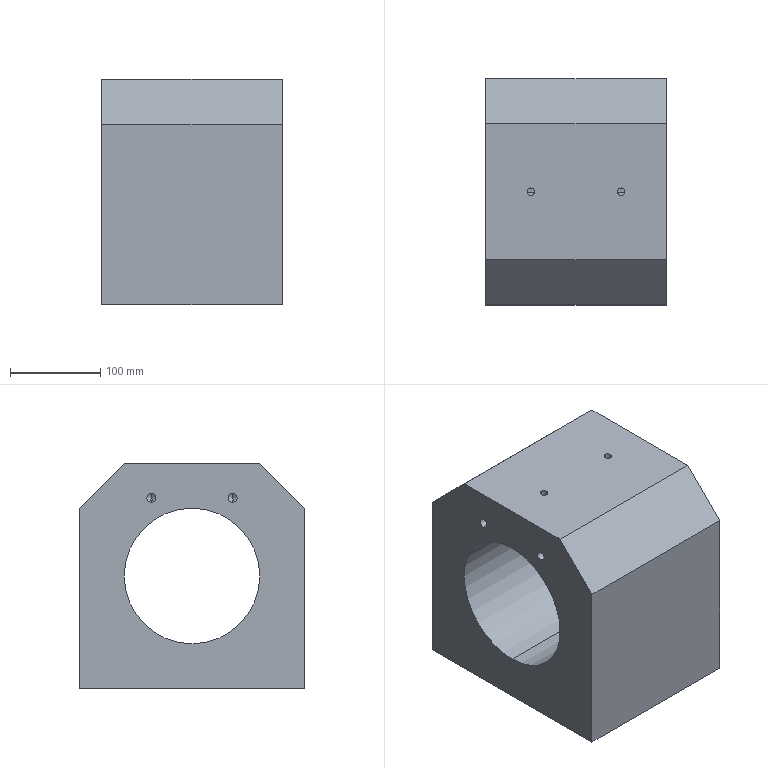Component | SolidWorks | BearingHousing-1_BearingHousing-1 | 1 solid | 30 faces | box 200 x 250 x 250 mm | volume 8448175 mm3 | cylinder 14 | cone 8 | plane 8 | commonest cylinder face diameters 10.2 x8 8.5 x4 150 x2 | material Plain Carbon Steel
STEP:
#1=COLOUR_RGB('',0.7922,0.8196,0.9333);
#2=FILL_AREA_STYLE_COLOUR('',#1);
#3=FILL_AREA_STYLE('',(#2));
#4=SURFACE_STYLE_FILL_AREA(#3);
#5=SURFACE_SIDE_STYLE('',(#4));
#6=SURFACE_STYLE_USAGE(.BOTH.,#5);
#7=PRESENTATION_STYLE_ASSIGNMENT((#6));
#8=CARTESIAN_POINT('',(420.858,129.202,273.246));
#9=VERTEX_POINT('',#8);
#10=CARTESIAN_POINT('',(420.858,129.202,273.647));
#11=VERTEX_POINT('',#10);
#12=CARTESIAN_POINT('',(420.858,129.202,273.447));
#13=DIRECTION('',(-1.,-0.,0.));
#14=DIRECTION('',(0.,0.,1.));
#15=AXIS2_PLACEMENT_3D('',#12,#13,#14);
#16=CIRCLE('',#15,0.2008);
#17=EDGE_CURVE('',#9,#11,#16,.T.);
#18=ORIENTED_EDGE('',*,*,#17,.F.);
#19=CARTESIAN_POINT('',(419.47,129.202,273.246));
#20=VERTEX_POINT('',#19);
#21=CARTESIAN_POINT('',(419.47,129.202,273.246));
#22=DIRECTION('',(-1.,-0.,0.));
#23=VECTOR('',#22,39.37);
#24=LINE('',#21,#23);
#25=EDGE_CURVE('',#9,#20,#24,.T.);
#26=ORIENTED_EDGE('',*,*,#25,.T.);
#27=CARTESIAN_POINT('',(419.47,129.202,273.647));
#28=VERTEX_POINT('',#27);
#29=CARTESIAN_POINT('',(419.47,129.202,273.447));
#30=DIRECTION('',(-1.,-0.,0.));
#31=DIRECTION('',(0.,0.,1.));
#32=AXIS2_PLACEMENT_3D('',#29,#30,#31);
#33=CIRCLE('',#32,0.2008);
#34=EDGE_CURVE('',#20,#28,#33,.T.);
#35=ORIENTED_EDGE('',*,*,#34,.T.);
#36=CARTESIAN_POINT('',(419.47,129.202,273.647));
#37=DIRECTION('',(-1.,-0.,0.));
#38=VECTOR('',#37,39.37);
#39=LINE('',#36,#38);
#40=EDGE_CURVE('',#11,#28,#39,.T.);
#41=ORIENTED_EDGE('',*,*,#40,.F.);
#42=EDGE_LOOP('',(#18,#26,#35,#41));
#43=FACE_OUTER_BOUND('',#42,.T.);
#44=CARTESIAN_POINT('',(419.47,129.202,273.447));
#45=DIRECTION('',(-1.,-0.,0.));
#46=DIRECTION('',(0.,0.,1.));
#47=AXIS2_PLACEMENT_3D('',#44,#45,#46);
#48=CYLINDRICAL_SURFACE('',#47,0.2008);
#49=ADVANCED_FACE('',(#43),#48,.F.);
#50=CARTESIAN_POINT('',(420.978,129.202,273.447));
#51=VERTEX_POINT('',#50);
#52=CARTESIAN_POINT('',(420.858,129.202,273.647));
#53=DIRECTION('',(-0.515,-0.,0.8572));
#54=VECTOR('',#53,39.37);
#55=LINE('',#52,#54);
#56=EDGE_CURVE('',#51,#11,#55,.T.);
#57=ORIENTED_EDGE('',*,*,#56,.F.);
#58=CARTESIAN_POINT('',(420.858,129.202,273.246));
#59=DIRECTION('',(-0.515,-0.,-0.8572));
#60=VECTOR('',#59,39.37);
#61=LINE('',#58,#60);
#62=EDGE_CURVE('',#51,#9,#61,.T.);
#63=ORIENTED_EDGE('',*,*,#62,.T.);
#64=ORIENTED_EDGE('',*,*,#17,.T.);
#65=EDGE_LOOP('',(#57,#63,#64));
#66=FACE_OUTER_BOUND('',#65,.T.);
#67=CARTESIAN_POINT('',(420.858,129.202,273.447));
#68=DIRECTION('',(-1.,-0.,0.));
#69=DIRECTION('',(0.,0.,1.));
#70=AXIS2_PLACEMENT_3D('',#67,#68,#69);
#71=CONICAL_SURFACE('',#70,0.2008,1.03);
#72=ADVANCED_FACE('',(#66),#71,.F.);
#73=CARTESIAN_POINT('',(420.858,125.659,273.246));
#74=VERTEX_POINT('',#73);
#75=CARTESIAN_POINT('',(420.858,125.659,273.647));
#76=VERTEX_POINT('',#75);
#77=CARTESIAN_POINT('',(420.858,125.659,273.447));
#78=DIRECTION('',(-1.,-0.,0.));
#79=DIRECTION('',(0.,0.,1.));
#80=AXIS2_PLACEMENT_3D('',#77,#78,#79);
#81=CIRCLE('',#80,0.2008);
#82=EDGE_CURVE('',#74,#76,#81,.T.);
#83=ORIENTED_EDGE('',*,*,#82,.F.);
#84=CARTESIAN_POINT('',(419.47,125.659,273.246));
#85=VERTEX_POINT('',#84);
#86=CARTESIAN_POINT('',(419.47,125.659,273.246));
#87=DIRECTION('',(-1.,-0.,0.));
#88=VECTOR('',#87,39.37);
#89=LINE('',#86,#88);
#90=EDGE_CURVE('',#74,#85,#89,.T.);
#91=ORIENTED_EDGE('',*,*,#90,.T.);
#92=CARTESIAN_POINT('',(419.47,125.659,273.647));
#93=VERTEX_POINT('',#92);
#94=CARTESIAN_POINT('',(419.47,125.659,273.447));
#95=DIRECTION('',(-1.,-0.,0.));
#96=DIRECTION('',(0.,0.,1.));
#97=AXIS2_PLACEMENT_3D('',#94,#95,#96);
#98=CIRCLE('',#97,0.2008);
#99=EDGE_CURVE('',#85,#93,#98,.T.);
#100=ORIENTED_EDGE('',*,*,#99,.T.);
#101=CARTESIAN_POINT('',(419.47,125.659,273.647));
#102=DIRECTION('',(-1.,-0.,0.));
#103=VECTOR('',#102,39.37);
#104=LINE('',#101,#103);
#105=EDGE_CURVE('',#76,#93,#104,.T.);
#106=ORIENTED_EDGE('',*,*,#105,.F.);
#107=EDGE_LOOP('',(#83,#91,#100,#106));
#108=FACE_OUTER_BOUND('',#107,.T.);
#109=CARTESIAN_POINT('',(419.47,125.659,273.447));
#110=DIRECTION('',(-1.,-0.,0.));
#111=DIRECTION('',(0.,0.,1.));
#112=AXIS2_PLACEMENT_3D('',#109,#110,#111);
#113=CYLINDRICAL_SURFACE('',#112,0.2008);
#114=ADVANCED_FACE('',(#108),#113,.F.);
#115=CARTESIAN_POINT('',(420.978,125.659,273.447));
#116=VERTEX_POINT('',#115);
#117=CARTESIAN_POINT('',(420.858,125.659,273.647));
#118=DIRECTION('',(-0.515,-0.,0.8572));
#119=VECTOR('',#118,39.37);
#120=LINE('',#117,#119);
#121=EDGE_CURVE('',#116,#76,#120,.T.);
#122=ORIENTED_EDGE('',*,*,#121,.F.);
#123=CARTESIAN_POINT('',(420.858,125.659,273.246));
#124=DIRECTION('',(-0.515,-0.,-0.8572));
#125=VECTOR('',#124,39.37);
#126=LINE('',#123,#125);
#127=EDGE_CURVE('',#116,#74,#126,.T.);
#128=ORIENTED_EDGE('',*,*,#127,.T.);
#129=ORIENTED_EDGE('',*,*,#82,.T.);
#130=EDGE_LOOP('',(#122,#128,#129));
#131=FACE_OUTER_BOUND('',#130,.T.);
#132=CARTESIAN_POINT('',(420.858,125.659,273.447));
#133=DIRECTION('',(-1.,-0.,0.));
#134=DIRECTION('',(0.,0.,1.));
#135=AXIS2_PLACEMENT_3D('',#132,#133,#134);
#136=CONICAL_SURFACE('',#135,0.2008,1.03);
#137=ADVANCED_FACE('',(#131),#136,.F.);
#138=CARTESIAN_POINT('',(425.956,125.659,273.529));
#139=VERTEX_POINT('',#138);
#140=CARTESIAN_POINT('',(425.956,125.659,273.128));
#141=VERTEX_POINT('',#140);
#142=CARTESIAN_POINT('',(425.956,125.659,273.328));
#143=DIRECTION('',(1.,0.,0.));
#144=DIRECTION('',(0.,0.,-1.));
#145=AXIS2_PLACEMENT_3D('',#142,#143,#144);
#146=CIRCLE('',#145,0.2008);
#147=EDGE_CURVE('',#139,#141,#146,.T.);
#148=ORIENTED_EDGE('',*,*,#147,.F.);
#149=CARTESIAN_POINT('',(427.344,125.659,273.529));
#150=VERTEX_POINT('',#149);
#151=CARTESIAN_POINT('',(427.344,125.659,273.529));
#152=DIRECTION('',(1.,0.,0.));
#153=VECTOR('',#152,39.37);
#154=LINE('',#151,#153);
#155=EDGE_CURVE('',#139,#150,#154,.T.);
#156=ORIENTED_EDGE('',*,*,#155,.T.);
#157=CARTESIAN_POINT('',(427.344,125.659,273.128));
#158=VERTEX_POINT('',#157);
#159=CARTESIAN_POINT('',(427.344,125.659,273.328));
#160=DIRECTION('',(1.,0.,0.));
#161=DIRECTION('',(0.,0.,-1.));
#162=AXIS2_PLACEMENT_3D('',#159,#160,#161);
#163=CIRCLE('',#162,0.2008);
#164=EDGE_CURVE('',#150,#158,#163,.T.);
#165=ORIENTED_EDGE('',*,*,#164,.T.);
#166=CARTESIAN_POINT('',(427.344,125.659,273.128));
#167=DIRECTION('',(1.,0.,0.));
#168=VECTOR('',#167,39.37);
#169=LINE('',#166,#168);
#170=EDGE_CURVE('',#141,#158,#169,.T.);
#171=ORIENTED_EDGE('',*,*,#170,.F.);
#172=EDGE_LOOP('',(#148,#156,#165,#171));
#173=FACE_OUTER_BOUND('',#172,.T.);
#174=CARTESIAN_POINT('',(427.344,125.659,273.328));
#175=DIRECTION('',(1.,0.,0.));
#176=DIRECTION('',(0.,0.,-1.));
#177=AXIS2_PLACEMENT_3D('',#174,#175,#176);
#178=CYLINDRICAL_SURFACE('',#177,0.2008);
#179=ADVANCED_FACE('',(#173),#178,.F.);
#180=CARTESIAN_POINT('',(425.835,125.659,273.328));
#181=VERTEX_POINT('',#180);
#182=CARTESIAN_POINT('',(425.956,125.659,273.128));
#183=DIRECTION('',(0.515,0.,-0.8572));
#184=VECTOR('',#183,39.37);
#185=LINE('',#182,#184);
#186=EDGE_CURVE('',#181,#141,#185,.T.);
#187=ORIENTED_EDGE('',*,*,#186,.F.);
#188=CARTESIAN_POINT('',(425.956,125.659,273.529));
#189=DIRECTION('',(0.515,0.,0.8572));
#190=VECTOR('',#189,39.37);
#191=LINE('',#188,#190);
#192=EDGE_CURVE('',#181,#139,#191,.T.);
#193=ORIENTED_EDGE('',*,*,#192,.T.);
#194=ORIENTED_EDGE('',*,*,#147,.T.);
#195=EDGE_LOOP('',(#187,#193,#194));
#196=FACE_OUTER_BOUND('',#195,.T.);
#197=CARTESIAN_POINT('',(425.956,125.659,273.328));
#198=DIRECTION('',(1.,0.,0.));
#199=DIRECTION('',(0.,0.,-1.));
#200=AXIS2_PLACEMENT_3D('',#197,#198,#199);
#201=CONICAL_SURFACE('',#200,0.2008,1.03);
#202=ADVANCED_FACE('',(#196),#201,.F.);
#203=CARTESIAN_POINT('',(425.956,129.202,273.529));
#204=VERTEX_POINT('',#203);
#205=CARTESIAN_POINT('',(425.956,129.202,273.128));
#206=VERTEX_POINT('',#205);
#207=CARTESIAN_POINT('',(425.956,129.202,273.328));
#208=DIRECTION('',(1.,0.,0.));
#209=DIRECTION('',(0.,0.,-1.));
#210=AXIS2_PLACEMENT_3D('',#207,#208,#209);
#211=CIRCLE('',#210,0.2008);
#212=EDGE_CURVE('',#204,#206,#211,.T.);
#213=ORIENTED_EDGE('',*,*,#212,.F.);
#214=CARTESIAN_POINT('',(427.344,129.202,273.529));
#215=VERTEX_POINT('',#214);
#216=CARTESIAN_POINT('',(427.344,129.202,273.529));
#217=DIRECTION('',(1.,0.,0.));
#218=VECTOR('',#217,39.37);
#219=LINE('',#216,#218);
#220=EDGE_CURVE('',#204,#215,#219,.T.);
#221=ORIENTED_EDGE('',*,*,#220,.T.);
#222=CARTESIAN_POINT('',(427.344,129.202,273.128));
#223=VERTEX_POINT('',#222);
#224=CARTESIAN_POINT('',(427.344,129.202,273.328));
#225=DIRECTION('',(1.,0.,0.));
#226=DIRECTION('',(0.,0.,-1.));
#227=AXIS2_PLACEMENT_3D('',#224,#225,#226);
#228=CIRCLE('',#227,0.2008);
#229=EDGE_CURVE('',#215,#223,#228,.T.);
#230=ORIENTED_EDGE('',*,*,#229,.T.);
#231=CARTESIAN_POINT('',(427.344,129.202,273.128));
#232=DIRECTION('',(1.,0.,0.));
#233=VECTOR('',#232,39.37);
#234=LINE('',#231,#233);
#235=EDGE_CURVE('',#206,#223,#234,.T.);
#236=ORIENTED_EDGE('',*,*,#235,.F.);
#237=EDGE_LOOP('',(#213,#221,#230,#236));
#238=FACE_OUTER_BOUND('',#237,.T.);
#239=CARTESIAN_POINT('',(427.344,129.202,273.328));
#240=DIRECTION('',(1.,0.,0.));
#241=DIRECTION('',(0.,0.,-1.));
#242=AXIS2_PLACEMENT_3D('',#239,#240,#241);
#243=CYLINDRICAL_SURFACE('',#242,0.2008);
#244=ADVANCED_FACE('',(#238),#243,.F.);
#245=CARTESIAN_POINT('',(425.835,129.202,273.328));
#246=VERTEX_POINT('',#245);
#247=CARTESIAN_POINT('',(425.956,129.202,273.128));
#248=DIRECTION('',(0.515,0.,-0.8572));
#249=VECTOR('',#248,39.37);
#250=LINE('',#247,#249);
#251=EDGE_CURVE('',#246,#206,#250,.T.);
#252=ORIENTED_EDGE('',*,*,#251,.F.);
#253=CARTESIAN_POINT('',(425.956,129.202,273.529));
#254=DIRECTION('',(0.515,0.,0.8572));
#255=VECTOR('',#254,39.37);
#256=LINE('',#253,#255);
#257=EDGE_CURVE('',#246,#204,#256,.T.);
#258=ORIENTED_EDGE('',*,*,#257,.T.);
#259=ORIENTED_EDGE('',*,*,#212,.T.);
#260=EDGE_LOOP('',(#252,#258,#259));
#261=FACE_OUTER_BOUND('',#260,.T.);
#262=CARTESIAN_POINT('',(425.956,129.202,273.328));
#263=DIRECTION('',(1.,0.,0.));
#264=DIRECTION('',(0.,0.,-1.));
#265=AXIS2_PLACEMENT_3D('',#262,#263,#264);
#266=CONICAL_SURFACE('',#265,0.2008,1.03);
#267=ADVANCED_FACE('',(#261),#266,.F.);
#268=CARTESIAN_POINT('',(421.606,127.43,272.994));
#269=VERTEX_POINT('',#268);
#270=CARTESIAN_POINT('',(421.438,127.263,272.989));
#271=VERTEX_POINT('',#270);
#272=CARTESIAN_POINT('',(421.606,127.43,272.994));
#273=CARTESIAN_POINT('',(421.606,127.42,272.994));
#274=CARTESIAN_POINT('',(421.605,127.408,272.994));
#275=CARTESIAN_POINT('',(421.6,127.387,272.994));
#276=CARTESIAN_POINT('',(421.597,127.377,272.993));
#277=CARTESIAN_POINT('',(421.589,127.356,272.993));
#278=CARTESIAN_POINT('',(421.584,127.346,272.993));
#279=CARTESIAN_POINT('',(421.571,127.328,272.992));
#280=CARTESIAN_POINT('',(421.565,127.32,272.992));
#281=CARTESIAN_POINT('',(421.549,127.304,272.991));
#282=CARTESIAN_POINT('',(421.54,127.297,272.991));
#283=CARTESIAN_POINT('',(421.522,127.285,272.99));
#284=CARTESIAN_POINT('',(421.513,127.28,272.99));
#285=CARTESIAN_POINT('',(421.492,127.272,272.99));
#286=CARTESIAN_POINT('',(421.482,127.268,272.989));
#287=CARTESIAN_POINT('',(421.46,127.264,272.989));
#288=CARTESIAN_POINT('',(421.449,127.263,272.989));
#289=CARTESIAN_POINT('',(421.438,127.263,272.989));
#290=B_SPLINE_CURVE_WITH_KNOTS('',3,(#272,#273,#274,#275,#276,#277,#278,#279,#280,#281,#282,#283,#284,#285,#286,#287,#288,#289),.UNSPECIFIED.,.F.,.F.,(4,2,2,2,2,2,2,2,4),(0.006647,0.007477,0.008307,0.009138,0.009968,0.0108,0.01163,0.01246,0.01329),.UNSPECIFIED.);
#291=EDGE_CURVE('',#269,#271,#290,.T.);
#292=ORIENTED_EDGE('',*,*,#291,.T.);
#293=CARTESIAN_POINT('',(421.438,127.263,274.962));
#294=VERTEX_POINT('',#293);
#295=CARTESIAN_POINT('',(421.438,127.263,274.962));
#296=DIRECTION('',(0.,0.,1.));
#297=VECTOR('',#296,39.37);
#298=LINE('',#295,#297);
#299=EDGE_CURVE('',#271,#294,#298,.T.);
#300=ORIENTED_EDGE('',*,*,#299,.T.);
#301=CARTESIAN_POINT('',(421.438,127.598,274.962));
#302=VERTEX_POINT('',#301);
#303=CARTESIAN_POINT('',(421.438,127.43,274.962));
#304=DIRECTION('',(0.,0.,1.));
#305=DIRECTION('',(0.,1.,0.));
#306=AXIS2_PLACEMENT_3D('',#303,#304,#305);
#307=CIRCLE('',#306,0.1673);
#308=EDGE_CURVE('',#294,#302,#307,.T.);
#309=ORIENTED_EDGE('',*,*,#308,.T.);
#310=CARTESIAN_POINT('',(421.438,127.598,272.989));
#311=VERTEX_POINT('',#310);
#312=CARTESIAN_POINT('',(421.438,127.598,274.962));
#313=DIRECTION('',(0.,0.,1.));
#314=VECTOR('',#313,39.37);
#315=LINE('',#312,#314);
#316=EDGE_CURVE('',#311,#302,#315,.T.);
#317=ORIENTED_EDGE('',*,*,#316,.F.);
#318=CARTESIAN_POINT('',(421.438,127.598,272.989));
#319=CARTESIAN_POINT('',(421.449,127.598,272.989));
#320=CARTESIAN_POINT('',(421.46,127.597,272.989));
#321=CARTESIAN_POINT('',(421.482,127.592,272.989));
#322=CARTESIAN_POINT('',(421.492,127.589,272.99));
#323=CARTESIAN_POINT('',(421.513,127.581,272.99));
#324=CARTESIAN_POINT('',(421.522,127.576,272.99));
#325=CARTESIAN_POINT('',(421.54,127.563,272.991));
#326=CARTESIAN_POINT('',(421.549,127.556,272.991));
#327=CARTESIAN_POINT('',(421.564,127.541,272.992));
#328=CARTESIAN_POINT('',(421.571,127.533,272.992));
#329=CARTESIAN_POINT('',(421.584,127.514,272.993));
#330=CARTESIAN_POINT('',(421.589,127.505,272.993));
#331=CARTESIAN_POINT('',(421.597,127.484,272.993));
#332=CARTESIAN_POINT('',(421.6,127.474,272.994));
#333=CARTESIAN_POINT('',(421.605,127.452,272.994));
#334=CARTESIAN_POINT('',(421.606,127.441,272.994));
#335=CARTESIAN_POINT('',(421.606,127.43,272.994));
#336=B_SPLINE_CURVE_WITH_KNOTS('',3,(#318,#319,#320,#321,#322,#323,#324,#325,#326,#327,#328,#329,#330,#331,#332,#333,#334,#335),.UNSPECIFIED.,.F.,.F.,(4,2,2,2,2,2,2,2,4),(0.,0.0008308,0.001662,0.002492,0.003323,0.004154,0.004985,0.005816,0.006647),.UNSPECIFIED.);
#337=EDGE_CURVE('',#311,#269,#336,.T.);
#338=ORIENTED_EDGE('',*,*,#337,.T.);
#339=EDGE_LOOP('',(#292,#300,#309,#317,#338));
#340=FACE_OUTER_BOUND('',#339,.T.);
#341=CARTESIAN_POINT('',(421.438,127.43,274.962));
#342=DIRECTION('',(0.,0.,1.));
#343=DIRECTION('',(0.,1.,0.));
#344=AXIS2_PLACEMENT_3D('',#341,#342,#343);
#345=CYLINDRICAL_SURFACE('',#344,0.1673);
#346=ADVANCED_FACE('',(#340),#345,.F.);
#347=CARTESIAN_POINT('',(425.543,127.43,272.994));
#348=VERTEX_POINT('',#347);
#349=CARTESIAN_POINT('',(425.375,127.263,272.989));
#350=VERTEX_POINT('',#349);
#351=CARTESIAN_POINT('',(425.543,127.43,272.994));
#352=CARTESIAN_POINT('',(425.543,127.42,272.994));
#353=CARTESIAN_POINT('',(425.542,127.408,272.994));
#354=CARTESIAN_POINT('',(425.537,127.387,272.994));
#355=CARTESIAN_POINT('',(425.534,127.377,272.993));
#356=CARTESIAN_POINT('',(425.526,127.356,272.993));
#357=CARTESIAN_POINT('',(425.521,127.346,272.993));
#358=CARTESIAN_POINT('',(425.508,127.328,272.992));
#359=CARTESIAN_POINT('',(425.502,127.32,272.992));
#360=CARTESIAN_POINT('',(425.486,127.304,272.991));
#361=CARTESIAN_POINT('',(425.477,127.297,272.991));
#362=CARTESIAN_POINT('',(425.459,127.285,272.99));
#363=CARTESIAN_POINT('',(425.45,127.28,272.99));
#364=CARTESIAN_POINT('',(425.429,127.272,272.99));
#365=CARTESIAN_POINT('',(425.419,127.268,272.989));
#366=CARTESIAN_POINT('',(425.397,127.264,272.989));
#367=CARTESIAN_POINT('',(425.386,127.263,272.989));
#368=CARTESIAN_POINT('',(425.375,127.263,272.989));
#369=B_SPLINE_CURVE_WITH_KNOTS('',3,(#351,#352,#353,#354,#355,#356,#357,#358,#359,#360,#361,#362,#363,#364,#365,#366,#367,#368),.UNSPECIFIED.,.F.,.F.,(4,2,2,2,2,2,2,2,4),(0.006647,0.007477,0.008307,0.009138,0.009968,0.0108,0.01163,0.01246,0.01329),.UNSPECIFIED.);
#370=EDGE_CURVE('',#348,#350,#369,.T.);
#371=ORIENTED_EDGE('',*,*,#370,.T.);
#372=CARTESIAN_POINT('',(425.375,127.263,274.962));
#373=VERTEX_POINT('',#372);
#374=CARTESIAN_POINT('',(425.375,127.263,274.962));
#375=DIRECTION('',(0.,0.,1.));
#376=VECTOR('',#375,39.37);
#377=LINE('',#374,#376);
#378=EDGE_CURVE('',#350,#373,#377,.T.);
#379=ORIENTED_EDGE('',*,*,#378,.T.);
#380=CARTESIAN_POINT('',(425.375,127.598,274.962));
#381=VERTEX_POINT('',#380);
#382=CARTESIAN_POINT('',(425.375,127.43,274.962));
#383=DIRECTION('',(0.,0.,1.));
#384=DIRECTION('',(0.,1.,0.));
#385=AXIS2_PLACEMENT_3D('',#382,#383,#384);
#386=CIRCLE('',#385,0.1673);
#387=EDGE_CURVE('',#373,#381,#386,.T.);
#388=ORIENTED_EDGE('',*,*,#387,.T.);
#389=CARTESIAN_POINT('',(425.375,127.598,272.989));
#390=VERTEX_POINT('',#389);
#391=CARTESIAN_POINT('',(425.375,127.598,274.962));
#392=DIRECTION('',(0.,0.,1.));
#393=VECTOR('',#392,39.37);
#394=LINE('',#391,#393);
#395=EDGE_CURVE('',#390,#381,#394,.T.);
#396=ORIENTED_EDGE('',*,*,#395,.F.);
#397=CARTESIAN_POINT('',(425.375,127.598,272.989));
#398=CARTESIAN_POINT('',(425.386,127.598,272.989));
#399=CARTESIAN_POINT('',(425.397,127.597,272.989));
#400=CARTESIAN_POINT('',(425.419,127.592,272.989));
#401=CARTESIAN_POINT('',(425.429,127.589,272.99));
#402=CARTESIAN_POINT('',(425.45,127.581,272.99));
#403=CARTESIAN_POINT('',(425.459,127.576,272.99));
#404=CARTESIAN_POINT('',(425.477,127.563,272.991));
#405=CARTESIAN_POINT('',(425.486,127.556,272.991));
#406=CARTESIAN_POINT('',(425.501,127.541,272.992));
#407=CARTESIAN_POINT('',(425.508,127.533,272.992));
#408=CARTESIAN_POINT('',(425.521,127.514,272.993));
#409=CARTESIAN_POINT('',(425.526,127.505,272.993));
#410=CARTESIAN_POINT('',(425.534,127.484,272.993));
#411=CARTESIAN_POINT('',(425.537,127.474,272.994));
#412=CARTESIAN_POINT('',(425.542,127.452,272.994));
#413=CARTESIAN_POINT('',(425.543,127.441,272.994));
#414=CARTESIAN_POINT('',(425.543,127.43,272.994));
#415=B_SPLINE_CURVE_WITH_KNOTS('',3,(#397,#398,#399,#400,#401,#402,#403,#404,#405,#406,#407,#408,#409,#410,#411,#412,#413,#414),.UNSPECIFIED.,.F.,.F.,(4,2,2,2,2,2,2,2,4),(0.,0.0008308,0.001662,0.002492,0.003323,0.004154,0.004985,0.005816,0.006647),.UNSPECIFIED.);
#416=EDGE_CURVE('',#390,#348,#415,.T.);
#417=ORIENTED_EDGE('',*,*,#416,.T.);
#418=EDGE_LOOP('',(#371,#379,#388,#396,#417));
#419=FACE_OUTER_BOUND('',#418,.T.);
#420=CARTESIAN_POINT('',(425.375,127.43,274.962));
#421=DIRECTION('',(0.,0.,1.));
#422=DIRECTION('',(0.,1.,0.));
#423=AXIS2_PLACEMENT_3D('',#420,#421,#422);
#424=CYLINDRICAL_SURFACE('',#423,0.1673);
#425=ADVANCED_FACE('',(#419),#424,.F.);
#426=CARTESIAN_POINT('',(419.47,127.43,267.088));
#427=VERTEX_POINT('',#426);
#428=CARTESIAN_POINT('',(419.47,127.43,272.994));
#429=VERTEX_POINT('',#428);
#430=CARTESIAN_POINT('',(419.47,127.43,270.041));
#431=DIRECTION('',(-1.,-0.,0.));
#432=DIRECTION('',(0.,0.,1.));
#433=AXIS2_PLACEMENT_3D('',#430,#431,#432);
#434=CIRCLE('',#433,2.953);
#435=EDGE_CURVE('',#427,#429,#434,.T.);
#436=ORIENTED_EDGE('',*,*,#435,.T.);
#437=CARTESIAN_POINT('',(421.271,127.43,272.994));
#438=VERTEX_POINT('',#437);
#439=CARTESIAN_POINT('',(419.47,127.43,272.994));
#440=DIRECTION('',(1.,0.,0.));
#441=VECTOR('',#440,39.37);
#442=LINE('',#439,#441);
#443=EDGE_CURVE('',#429,#438,#442,.T.);
#444=ORIENTED_EDGE('',*,*,#443,.T.);
#445=CARTESIAN_POINT('',(421.438,127.263,272.989));
#446=CARTESIAN_POINT('',(421.427,127.263,272.989));
#447=CARTESIAN_POINT('',(421.417,127.264,272.989));
#448=CARTESIAN_POINT('',(421.395,127.268,272.989));
#449=CARTESIAN_POINT('',(421.384,127.272,272.99));
#450=CARTESIAN_POINT('',(421.364,127.28,272.99));
#451=CARTESIAN_POINT('',(421.355,127.285,272.99));
#452=CARTESIAN_POINT('',(421.336,127.297,272.991));
#453=CARTESIAN_POINT('',(421.328,127.304,272.991));
#454=CARTESIAN_POINT('',(421.312,127.32,272.992));
#455=CARTESIAN_POINT('',(421.305,127.328,272.992));
#456=CARTESIAN_POINT('',(421.293,127.347,272.993));
#457=CARTESIAN_POINT('',(421.288,127.356,272.993));
#458=CARTESIAN_POINT('',(421.28,127.376,272.993));
#459=CARTESIAN_POINT('',(421.276,127.387,272.994));
#460=CARTESIAN_POINT('',(421.272,127.409,272.994));
#461=CARTESIAN_POINT('',(421.271,127.419,272.994));
#462=CARTESIAN_POINT('',(421.271,127.43,272.994));
#463=B_SPLINE_CURVE_WITH_KNOTS('',3,(#445,#446,#447,#448,#449,#450,#451,#452,#453,#454,#455,#456,#457,#458,#459,#460,#461,#462),.UNSPECIFIED.,.F.,.F.,(4,2,2,2,2,2,2,2,4),(0.01329,0.01412,0.01495,0.01578,0.01661,0.01744,0.01828,0.01911,0.01994),.UNSPECIFIED.);
#464=EDGE_CURVE('',#271,#438,#463,.T.);
#465=ORIENTED_EDGE('',*,*,#464,.F.);
#466=ORIENTED_EDGE('',*,*,#291,.F.);
#467=CARTESIAN_POINT('',(425.208,127.43,272.994));
#468=VERTEX_POINT('',#467);
#469=CARTESIAN_POINT('',(419.47,127.43,272.994));
#470=DIRECTION('',(1.,0.,0.));
#471=VECTOR('',#470,39.37);
#472=LINE('',#469,#471);
#473=EDGE_CURVE('',#269,#468,#472,.T.);
#474=ORIENTED_EDGE('',*,*,#473,.T.);
#475=CARTESIAN_POINT('',(425.375,127.263,272.989));
#476=CARTESIAN_POINT('',(425.364,127.263,272.989));
#477=CARTESIAN_POINT('',(425.354,127.264,272.989));
#478=CARTESIAN_POINT('',(425.332,127.268,272.989));
#479=CARTESIAN_POINT('',(425.321,127.272,272.99));
#480=CARTESIAN_POINT('',(425.301,127.28,272.99));
#481=CARTESIAN_POINT('',(425.292,127.285,272.99));
#482=CARTESIAN_POINT('',(425.273,127.297,272.991));
#483=CARTESIAN_POINT('',(425.265,127.304,272.991));
#484=CARTESIAN_POINT('',(425.249,127.32,272.992));
#485=CARTESIAN_POINT('',(425.242,127.328,272.992));
#486=CARTESIAN_POINT('',(425.23,127.347,272.993));
#487=CARTESIAN_POINT('',(425.225,127.356,272.993));
#488=CARTESIAN_POINT('',(425.217,127.376,272.993));
#489=CARTESIAN_POINT('',(425.213,127.387,272.994));
#490=CARTESIAN_POINT('',(425.209,127.409,272.994));
#491=CARTESIAN_POINT('',(425.208,127.419,272.994));
#492=CARTESIAN_POINT('',(425.208,127.43,272.994));
#493=B_SPLINE_CURVE_WITH_KNOTS('',3,(#475,#476,#477,#478,#479,#480,#481,#482,#483,#484,#485,#486,#487,#488,#489,#490,#491,#492),.UNSPECIFIED.,.F.,.F.,(4,2,2,2,2,2,2,2,4),(0.01329,0.01412,0.01495,0.01578,0.01661,0.01744,0.01828,0.01911,0.01994),.UNSPECIFIED.);
#494=EDGE_CURVE('',#350,#468,#493,.T.);
#495=ORIENTED_EDGE('',*,*,#494,.F.);
#496=ORIENTED_EDGE('',*,*,#370,.F.);
#497=CARTESIAN_POINT('',(427.344,127.43,272.994));
#498=VERTEX_POINT('',#497);
#499=CARTESIAN_POINT('',(419.47,127.43,272.994));
#500=DIRECTION('',(1.,0.,0.));
#501=VECTOR('',#500,39.37);
#502=LINE('',#499,#501);
#503=EDGE_CURVE('',#348,#498,#502,.T.);
#504=ORIENTED_EDGE('',*,*,#503,.T.);
#505=CARTESIAN_POINT('',(427.344,127.43,267.088));
#506=VERTEX_POINT('',#505);
#507=CARTESIAN_POINT('',(427.344,127.43,270.041));
#508=DIRECTION('',(-1.,-0.,0.));
#509=DIRECTION('',(0.,0.,1.));
#510=AXIS2_PLACEMENT_3D('',#507,#508,#509);
#511=CIRCLE('',#510,2.953);
#512=EDGE_CURVE('',#506,#498,#511,.T.);
#513=ORIENTED_EDGE('',*,*,#512,.F.);
#514=CARTESIAN_POINT('',(419.47,127.43,267.088));
#515=DIRECTION('',(1.,0.,0.));
#516=VECTOR('',#515,39.37);
#517=LINE('',#514,#516);
#518=EDGE_CURVE('',#427,#506,#517,.T.);
#519=ORIENTED_EDGE('',*,*,#518,.F.);
#520=EDGE_LOOP('',(#436,#444,#465,#466,#474,#495,#496,#504,#513,#519));
#521=FACE_OUTER_BOUND('',#520,.T.);
#522=CARTESIAN_POINT('',(419.47,127.43,270.041));
#523=DIRECTION('',(1.,0.,0.));
#524=DIRECTION('',(0.,0.,-1.));
#525=AXIS2_PLACEMENT_3D('',#522,#523,#524);
#526=CYLINDRICAL_SURFACE('',#525,2.953);
#527=ADVANCED_FACE('',(#521),#526,.F.);
#528=CARTESIAN_POINT('',(419.47,129.202,273.447));
#529=DIRECTION('',(-1.,-0.,0.));
#530=DIRECTION('',(0.,0.,1.));
#531=AXIS2_PLACEMENT_3D('',#528,#529,#530);
#532=CIRCLE('',#531,0.2008);
#533=EDGE_CURVE('',#28,#20,#532,.T.);
#534=ORIENTED_EDGE('',*,*,#533,.F.);
#535=ORIENTED_EDGE('',*,*,#34,.F.);
#536=EDGE_LOOP('',(#534,#535));
#537=FACE_BOUND('',#536,.T.);
#538=CARTESIAN_POINT('',(419.47,125.659,273.447));
#539=DIRECTION('',(-1.,-0.,0.));
#540=DIRECTION('',(0.,0.,1.));
#541=AXIS2_PLACEMENT_3D('',#538,#539,#540);
#542=CIRCLE('',#541,0.2008);
#543=EDGE_CURVE('',#93,#85,#542,.T.);
#544=ORIENTED_EDGE('',*,*,#543,.F.);
#545=ORIENTED_EDGE('',*,*,#99,.F.);
#546=EDGE_LOOP('',(#544,#545));
#547=FACE_BOUND('',#546,.T.);
#548=CARTESIAN_POINT('',(419.47,124.478,274.962));
#549=VERTEX_POINT('',#548);
#550=CARTESIAN_POINT('',(419.47,130.383,274.962));
#551=VERTEX_POINT('',#550);
#552=CARTESIAN_POINT('',(419.47,122.509,274.962));
#553=DIRECTION('',(-0.,1.,0.));
#554=VECTOR('',#553,39.37);
#555=LINE('',#552,#554);
#556=EDGE_CURVE('',#549,#551,#555,.T.);
#557=ORIENTED_EDGE('',*,*,#556,.T.);
#558=CARTESIAN_POINT('',(419.47,132.352,272.994));
#559=VERTEX_POINT('',#558);
#560=CARTESIAN_POINT('',(419.47,131.367,273.978));
#561=DIRECTION('',(-0.,0.7071,-0.7071));
#562=VECTOR('',#561,39.37);
#563=LINE('',#560,#562);
#564=EDGE_CURVE('',#551,#559,#563,.T.);
#565=ORIENTED_EDGE('',*,*,#564,.T.);
#566=CARTESIAN_POINT('',(419.47,132.352,265.12));
#567=VERTEX_POINT('',#566);
#568=CARTESIAN_POINT('',(419.47,132.352,265.12));
#569=DIRECTION('',(0.,0.,-1.));
#570=VECTOR('',#569,39.37);
#571=LINE('',#568,#570);
#572=EDGE_CURVE('',#559,#567,#571,.T.);
#573=ORIENTED_EDGE('',*,*,#572,.T.);
#574=CARTESIAN_POINT('',(419.47,122.509,265.12));
#575=VERTEX_POINT('',#574);
#576=CARTESIAN_POINT('',(419.47,122.509,265.12));
#577=DIRECTION('',(0.,-1.,0.));
#578=VECTOR('',#577,39.37);
#579=LINE('',#576,#578);
#580=EDGE_CURVE('',#567,#575,#579,.T.);
#581=ORIENTED_EDGE('',*,*,#580,.T.);
#582=CARTESIAN_POINT('',(419.47,122.509,272.994));
#583=VERTEX_POINT('',#582);
#584=CARTESIAN_POINT('',(419.47,122.509,265.12));
#585=DIRECTION('',(-0.,0.,1.));
#586=VECTOR('',#585,39.37);
#587=LINE('',#584,#586);
#588=EDGE_CURVE('',#575,#583,#587,.T.);
#589=ORIENTED_EDGE('',*,*,#588,.T.);
#590=CARTESIAN_POINT('',(419.47,118.572,269.057));
#591=DIRECTION('',(-0.,0.7071,0.7071));
#592=VECTOR('',#591,39.37);
#593=LINE('',#590,#592);
#594=EDGE_CURVE('',#583,#549,#593,.T.);
#595=ORIENTED_EDGE('',*,*,#594,.T.);
#596=EDGE_LOOP('',(#557,#565,#573,#581,#589,#595));
#597=FACE_OUTER_BOUND('',#596,.T.);
#598=ORIENTED_EDGE('',*,*,#435,.F.);
#599=CARTESIAN_POINT('',(419.47,127.43,270.041));
#600=DIRECTION('',(-1.,-0.,0.));
#601=DIRECTION('',(0.,0.,1.));
#602=AXIS2_PLACEMENT_3D('',#599,#600,#601);
#603=CIRCLE('',#602,2.953);
#604=EDGE_CURVE('',#429,#427,#603,.T.);
#605=ORIENTED_EDGE('',*,*,#604,.F.);
#606=EDGE_LOOP('',(#598,#605));
#607=FACE_BOUND('',#606,.T.);
#608=CARTESIAN_POINT('',(419.47,122.509,265.12));
#609=DIRECTION('',(-1.,-0.,0.));
#610=DIRECTION('',(0.,0.,1.));
#611=AXIS2_PLACEMENT_3D('',#608,#609,#610);
#612=PLANE('',#611);
#613=ADVANCED_FACE('',(#537,#547,#597,#607),#612,.T.);
#614=CARTESIAN_POINT('',(427.344,125.659,273.328));
#615=DIRECTION('',(1.,0.,0.));
#616=DIRECTION('',(0.,0.,-1.));
#617=AXIS2_PLACEMENT_3D('',#614,#615,#616);
#618=CIRCLE('',#617,0.2008);
#619=EDGE_CURVE('',#158,#150,#618,.T.);
#620=ORIENTED_EDGE('',*,*,#619,.F.);
#621=ORIENTED_EDGE('',*,*,#164,.F.);
#622=EDGE_LOOP('',(#620,#621));
#623=FACE_BOUND('',#622,.T.);
#624=CARTESIAN_POINT('',(427.344,129.202,273.328));
#625=DIRECTION('',(1.,0.,0.));
#626=DIRECTION('',(0.,0.,-1.));
#627=AXIS2_PLACEMENT_3D('',#624,#625,#626);
#628=CIRCLE('',#627,0.2008);
#629=EDGE_CURVE('',#223,#215,#628,.T.);
#630=ORIENTED_EDGE('',*,*,#629,.F.);
#631=ORIENTED_EDGE('',*,*,#229,.F.);
#632=EDGE_LOOP('',(#630,#631));
#633=FACE_BOUND('',#632,.T.);
#634=CARTESIAN_POINT('',(427.344,132.352,272.994));
#635=VERTEX_POINT('',#634);
#636=CARTESIAN_POINT('',(427.344,132.352,265.12));
#637=VERTEX_POINT('',#636);
#638=CARTESIAN_POINT('',(427.344,132.352,265.12));
#639=DIRECTION('',(0.,0.,-1.));
#640=VECTOR('',#639,39.37);
#641=LINE('',#638,#640);
#642=EDGE_CURVE('',#635,#637,#641,.T.);
#643=ORIENTED_EDGE('',*,*,#642,.F.);
#644=CARTESIAN_POINT('',(427.344,130.383,274.962));
#645=VERTEX_POINT('',#644);
#646=CARTESIAN_POINT('',(427.344,132.352,272.994));
#647=DIRECTION('',(0.,-0.7071,0.7071));
#648=VECTOR('',#647,39.37);
#649=LINE('',#646,#648);
#650=EDGE_CURVE('',#635,#645,#649,.T.);
#651=ORIENTED_EDGE('',*,*,#650,.T.);
#652=CARTESIAN_POINT('',(427.344,124.478,274.962));
#653=VERTEX_POINT('',#652);
#654=CARTESIAN_POINT('',(427.344,122.509,274.962));
#655=DIRECTION('',(-0.,1.,0.));
#656=VECTOR('',#655,39.37);
#657=LINE('',#654,#656);
#658=EDGE_CURVE('',#653,#645,#657,.T.);
#659=ORIENTED_EDGE('',*,*,#658,.F.);
#660=CARTESIAN_POINT('',(427.344,122.509,272.994));
#661=VERTEX_POINT('',#660);
#662=CARTESIAN_POINT('',(427.344,124.478,274.962));
#663=DIRECTION('',(0.,-0.7071,-0.7071));
#664=VECTOR('',#663,39.37);
#665=LINE('',#662,#664);
#666=EDGE_CURVE('',#653,#661,#665,.T.);
#667=ORIENTED_EDGE('',*,*,#666,.T.);
#668=CARTESIAN_POINT('',(427.344,122.509,265.12));
#669=VERTEX_POINT('',#668);
#670=CARTESIAN_POINT('',(427.344,122.509,265.12));
#671=DIRECTION('',(-0.,0.,1.));
#672=VECTOR('',#671,39.37);
#673=LINE('',#670,#672);
#674=EDGE_CURVE('',#669,#661,#673,.T.);
#675=ORIENTED_EDGE('',*,*,#674,.F.);
#676=CARTESIAN_POINT('',(427.344,122.509,265.12));
#677=DIRECTION('',(0.,-1.,0.));
#678=VECTOR('',#677,39.37);
#679=LINE('',#676,#678);
#680=EDGE_CURVE('',#637,#669,#679,.T.);
#681=ORIENTED_EDGE('',*,*,#680,.F.);
#682=EDGE_LOOP('',(#643,#651,#659,#667,#675,#681));
#683=FACE_OUTER_BOUND('',#682,.T.);
#684=ORIENTED_EDGE('',*,*,#512,.T.);
#685=CARTESIAN_POINT('',(427.344,127.43,270.041));
#686=DIRECTION('',(-1.,-0.,0.));
#687=DIRECTION('',(0.,0.,1.));
#688=AXIS2_PLACEMENT_3D('',#685,#686,#687);
#689=CIRCLE('',#688,2.953);
#690=EDGE_CURVE('',#498,#506,#689,.T.);
#691=ORIENTED_EDGE('',*,*,#690,.T.);
#692=EDGE_LOOP('',(#684,#691));
#693=FACE_BOUND('',#692,.T.);
#694=CARTESIAN_POINT('',(427.344,122.509,265.12));
#695=DIRECTION('',(-1.,-0.,0.));
#696=DIRECTION('',(0.,0.,1.));
#697=AXIS2_PLACEMENT_3D('',#694,#695,#696);
#698=PLANE('',#697);
#699=ADVANCED_FACE('',(#623,#633,#683,#693),#698,.F.);
#700=ORIENTED_EDGE('',*,*,#674,.T.);
#701=CARTESIAN_POINT('',(419.47,122.509,272.994));
#702=DIRECTION('',(-1.,-0.,0.));
#703=VECTOR('',#702,39.37);
#704=LINE('',#701,#703);
#705=EDGE_CURVE('',#661,#583,#704,.T.);
#706=ORIENTED_EDGE('',*,*,#705,.T.);
#707=ORIENTED_EDGE('',*,*,#588,.F.);
#708=CARTESIAN_POINT('',(419.47,122.509,265.12));
#709=DIRECTION('',(1.,0.,0.));
#710=VECTOR('',#709,39.37);
#711=LINE('',#708,#710);
#712=EDGE_CURVE('',#575,#669,#711,.T.);
#713=ORIENTED_EDGE('',*,*,#712,.T.);
#714=EDGE_LOOP('',(#700,#706,#707,#713));
#715=FACE_OUTER_BOUND('',#714,.T.);
#716=CARTESIAN_POINT('',(419.47,122.509,265.12));
#717=DIRECTION('',(-0.,1.,-0.));
#718=DIRECTION('',(0.,-0.,-1.));
#719=AXIS2_PLACEMENT_3D('',#716,#717,#718);
#720=PLANE('',#719);
#721=ADVANCED_FACE('',(#715),#720,.F.);
#722=CARTESIAN_POINT('',(421.438,127.43,274.962));
#723=DIRECTION('',(0.,0.,1.));
#724=DIRECTION('',(0.,1.,0.));
#725=AXIS2_PLACEMENT_3D('',#722,#723,#724);
#726=CIRCLE('',#725,0.1673);
#727=EDGE_CURVE('',#302,#294,#726,.T.);
#728=ORIENTED_EDGE('',*,*,#727,.F.);
#729=ORIENTED_EDGE('',*,*,#308,.F.);
#730=EDGE_LOOP('',(#728,#729));
#731=FACE_BOUND('',#730,.T.);
#732=CARTESIAN_POINT('',(425.375,127.43,274.962));
#733=DIRECTION('',(0.,0.,1.));
#734=DIRECTION('',(0.,1.,0.));
#735=AXIS2_PLACEMENT_3D('',#732,#733,#734);
#736=CIRCLE('',#735,0.1673);
#737=EDGE_CURVE('',#381,#373,#736,.T.);
#738=ORIENTED_EDGE('',*,*,#737,.F.);
#739=ORIENTED_EDGE('',*,*,#387,.F.);
#740=EDGE_LOOP('',(#738,#739));
#741=FACE_BOUND('',#740,.T.);
#742=ORIENTED_EDGE('',*,*,#658,.T.);
#743=CARTESIAN_POINT('',(419.47,130.383,274.962));
#744=DIRECTION('',(-1.,-0.,0.));
#745=VECTOR('',#744,39.37);
#746=LINE('',#743,#745);
#747=EDGE_CURVE('',#645,#551,#746,.T.);
#748=ORIENTED_EDGE('',*,*,#747,.T.);
#749=ORIENTED_EDGE('',*,*,#556,.F.);
#750=CARTESIAN_POINT('',(419.47,124.478,274.962));
#751=DIRECTION('',(1.,0.,0.));
#752=VECTOR('',#751,39.37);
#753=LINE('',#750,#752);
#754=EDGE_CURVE('',#549,#653,#753,.T.);
#755=ORIENTED_EDGE('',*,*,#754,.T.);
#756=EDGE_LOOP('',(#742,#748,#749,#755));
#757=FACE_OUTER_BOUND('',#756,.T.);
#758=CARTESIAN_POINT('',(419.47,122.509,274.962));
#759=DIRECTION('',(0.,0.,-1.));
#760=DIRECTION('',(0.,-1.,0.));
#761=AXIS2_PLACEMENT_3D('',#758,#759,#760);
#762=PLANE('',#761);
#763=ADVANCED_FACE('',(#731,#741,#757),#762,.F.);
#764=ORIENTED_EDGE('',*,*,#572,.F.);
#765=CARTESIAN_POINT('',(419.47,132.352,272.994));
#766=DIRECTION('',(1.,0.,0.));
#767=VECTOR('',#766,39.37);
#768=LINE('',#765,#767);
#769=EDGE_CURVE('',#559,#635,#768,.T.);
#770=ORIENTED_EDGE('',*,*,#769,.T.);
#771=ORIENTED_EDGE('',*,*,#642,.T.);
#772=CARTESIAN_POINT('',(419.47,132.352,265.12));
#773=DIRECTION('',(1.,0.,0.));
#774=VECTOR('',#773,39.37);
#775=LINE('',#772,#774);
#776=EDGE_CURVE('',#567,#637,#775,.T.);
#777=ORIENTED_EDGE('',*,*,#776,.F.);
#778=EDGE_LOOP('',(#764,#770,#771,#777));
#779=FACE_OUTER_BOUND('',#778,.T.);
#780=CARTESIAN_POINT('',(419.47,132.352,265.12));
#781=DIRECTION('',(0.,-1.,0.));
#782=DIRECTION('',(0.,0.,1.));
#783=AXIS2_PLACEMENT_3D('',#780,#781,#782);
#784=PLANE('',#783);
#785=ADVANCED_FACE('',(#779),#784,.F.);
#786=ORIENTED_EDGE('',*,*,#680,.T.);
#787=ORIENTED_EDGE('',*,*,#712,.F.);
#788=ORIENTED_EDGE('',*,*,#580,.F.);
#789=ORIENTED_EDGE('',*,*,#776,.T.);
#790=EDGE_LOOP('',(#786,#787,#788,#789));
#791=FACE_OUTER_BOUND('',#790,.T.);
#792=CARTESIAN_POINT('',(419.47,122.509,265.12));
#793=DIRECTION('',(0.,0.,1.));
#794=DIRECTION('',(-0.,1.,0.));
#795=AXIS2_PLACEMENT_3D('',#792,#793,#794);
#796=PLANE('',#795);
#797=ADVANCED_FACE('',(#791),#796,.F.);
#798=ORIENTED_EDGE('',*,*,#443,.F.);
#799=ORIENTED_EDGE('',*,*,#604,.T.);
#800=ORIENTED_EDGE('',*,*,#518,.T.);
#801=ORIENTED_EDGE('',*,*,#690,.F.);
#802=ORIENTED_EDGE('',*,*,#503,.F.);
#803=ORIENTED_EDGE('',*,*,#416,.F.);
#804=CARTESIAN_POINT('',(425.208,127.43,272.994));
#805=CARTESIAN_POINT('',(425.208,127.441,272.994));
#806=CARTESIAN_POINT('',(425.209,127.452,272.994));
#807=CARTESIAN_POINT('',(425.213,127.474,272.994));
#808=CARTESIAN_POINT('',(425.217,127.484,272.993));
#809=CARTESIAN_POINT('',(425.225,127.505,272.993));
#810=CARTESIAN_POINT('',(425.23,127.514,272.993));
#811=CARTESIAN_POINT('',(425.242,127.532,272.992));
#812=CARTESIAN_POINT('',(425.249,127.541,272.992));
#813=CARTESIAN_POINT('',(425.265,127.556,272.991));
#814=CARTESIAN_POINT('',(425.273,127.563,272.991));
#815=CARTESIAN_POINT('',(425.291,127.576,272.99));
#816=CARTESIAN_POINT('',(425.301,127.581,272.99));
#817=CARTESIAN_POINT('',(425.321,127.589,272.99));
#818=CARTESIAN_POINT('',(425.332,127.592,272.989));
#819=CARTESIAN_POINT('',(425.353,127.597,272.989));
#820=CARTESIAN_POINT('',(425.364,127.598,272.989));
#821=CARTESIAN_POINT('',(425.375,127.598,272.989));
#822=B_SPLINE_CURVE_WITH_KNOTS('',3,(#804,#805,#806,#807,#808,#809,#810,#811,#812,#813,#814,#815,#816,#817,#818,#819,#820,#821),.UNSPECIFIED.,.F.,.F.,(4,2,2,2,2,2,2,2,4),(0.01994,0.02077,0.0216,0.02243,0.02326,0.02409,0.02492,0.02575,0.02658),.UNSPECIFIED.);
#823=EDGE_CURVE('',#468,#390,#822,.T.);
#824=ORIENTED_EDGE('',*,*,#823,.F.);
#825=ORIENTED_EDGE('',*,*,#473,.F.);
#826=ORIENTED_EDGE('',*,*,#337,.F.);
#827=CARTESIAN_POINT('',(421.271,127.43,272.994));
#828=CARTESIAN_POINT('',(421.271,127.441,272.994));
#829=CARTESIAN_POINT('',(421.272,127.452,272.994));
#830=CARTESIAN_POINT('',(421.276,127.474,272.994));
#831=CARTESIAN_POINT('',(421.28,127.484,272.993));
#832=CARTESIAN_POINT('',(421.288,127.505,272.993));
#833=CARTESIAN_POINT('',(421.293,127.514,272.993));
#834=CARTESIAN_POINT('',(421.305,127.532,272.992));
#835=CARTESIAN_POINT('',(421.312,127.541,272.992));
#836=CARTESIAN_POINT('',(421.328,127.556,272.991));
#837=CARTESIAN_POINT('',(421.336,127.563,272.991));
#838=CARTESIAN_POINT('',(421.354,127.576,272.99));
#839=CARTESIAN_POINT('',(421.364,127.581,272.99));
#840=CARTESIAN_POINT('',(421.384,127.589,272.99));
#841=CARTESIAN_POINT('',(421.395,127.592,272.989));
#842=CARTESIAN_POINT('',(421.416,127.597,272.989));
#843=CARTESIAN_POINT('',(421.427,127.598,272.989));
#844=CARTESIAN_POINT('',(421.438,127.598,272.989));
#845=B_SPLINE_CURVE_WITH_KNOTS('',3,(#827,#828,#829,#830,#831,#832,#833,#834,#835,#836,#837,#838,#839,#840,#841,#842,#843,#844),.UNSPECIFIED.,.F.,.F.,(4,2,2,2,2,2,2,2,4),(0.01994,0.02077,0.0216,0.02243,0.02326,0.02409,0.02492,0.02575,0.02658),.UNSPECIFIED.);
#846=EDGE_CURVE('',#438,#311,#845,.T.);
#847=ORIENTED_EDGE('',*,*,#846,.F.);
#848=EDGE_LOOP('',(#798,#799,#800,#801,#802,#803,#824,#825,#826,#847));
#849=FACE_OUTER_BOUND('',#848,.T.);
#850=CARTESIAN_POINT('',(419.47,127.43,270.041));
#851=DIRECTION('',(1.,0.,0.));
#852=DIRECTION('',(0.,0.,-1.));
#853=AXIS2_PLACEMENT_3D('',#850,#851,#852);
#854=CYLINDRICAL_SURFACE('',#853,2.953);
#855=ADVANCED_FACE('',(#849),#854,.F.);
#856=ORIENTED_EDGE('',*,*,#564,.F.);
#857=ORIENTED_EDGE('',*,*,#747,.F.);
#858=ORIENTED_EDGE('',*,*,#650,.F.);
#859=ORIENTED_EDGE('',*,*,#769,.F.);
#860=EDGE_LOOP('',(#856,#857,#858,#859));
#861=FACE_OUTER_BOUND('',#860,.T.);
#862=CARTESIAN_POINT('',(419.47,132.352,272.994));
#863=DIRECTION('',(0.,-0.7071,-0.7071));
#864=DIRECTION('',(1.,0.,0.));
#865=AXIS2_PLACEMENT_3D('',#862,#863,#864);
#866=PLANE('',#865);
#867=ADVANCED_FACE('',(#861),#866,.F.);
#868=ORIENTED_EDGE('',*,*,#594,.F.);
#869=ORIENTED_EDGE('',*,*,#705,.F.);
#870=ORIENTED_EDGE('',*,*,#666,.F.);
#871=ORIENTED_EDGE('',*,*,#754,.F.);
#872=EDGE_LOOP('',(#868,#869,#870,#871));
#873=FACE_OUTER_BOUND('',#872,.T.);
#874=CARTESIAN_POINT('',(419.47,124.478,274.962));
#875=DIRECTION('',(-0.,0.7071,-0.7071));
#876=DIRECTION('',(1.,0.,0.));
#877=AXIS2_PLACEMENT_3D('',#874,#875,#876);
#878=PLANE('',#877);
#879=ADVANCED_FACE('',(#873),#878,.F.);
#880=ORIENTED_EDGE('',*,*,#378,.F.);
#881=ORIENTED_EDGE('',*,*,#494,.T.);
#882=ORIENTED_EDGE('',*,*,#823,.T.);
#883=ORIENTED_EDGE('',*,*,#395,.T.);
#884=ORIENTED_EDGE('',*,*,#737,.T.);
#885=EDGE_LOOP('',(#880,#881,#882,#883,#884));
#886=FACE_OUTER_BOUND('',#885,.T.);
#887=CARTESIAN_POINT('',(425.375,127.43,274.962));
#888=DIRECTION('',(0.,0.,1.));
#889=DIRECTION('',(0.,1.,0.));
#890=AXIS2_PLACEMENT_3D('',#887,#888,#889);
#891=CYLINDRICAL_SURFACE('',#890,0.1673);
#892=ADVANCED_FACE('',(#886),#891,.F.);
#893=ORIENTED_EDGE('',*,*,#299,.F.);
#894=ORIENTED_EDGE('',*,*,#464,.T.);
#895=ORIENTED_EDGE('',*,*,#846,.T.);
#896=ORIENTED_EDGE('',*,*,#316,.T.);
#897=ORIENTED_EDGE('',*,*,#727,.T.);
#898=EDGE_LOOP('',(#893,#894,#895,#896,#897));
#899=FACE_OUTER_BOUND('',#898,.T.);
#900=CARTESIAN_POINT('',(421.438,127.43,274.962));
#901=DIRECTION('',(0.,0.,1.));
#902=DIRECTION('',(0.,1.,0.));
#903=AXIS2_PLACEMENT_3D('',#900,#901,#902);
#904=CYLINDRICAL_SURFACE('',#903,0.1673);
#905=ADVANCED_FACE('',(#899),#904,.F.);
#906=ORIENTED_EDGE('',*,*,#257,.F.);
#907=ORIENTED_EDGE('',*,*,#251,.T.);
#908=CARTESIAN_POINT('',(425.956,129.202,273.328));
#909=DIRECTION('',(1.,0.,0.));
#910=DIRECTION('',(0.,0.,-1.));
#911=AXIS2_PLACEMENT_3D('',#908,#909,#910);
#912=CIRCLE('',#911,0.2008);
#913=EDGE_CURVE('',#206,#204,#912,.T.);
#914=ORIENTED_EDGE('',*,*,#913,.T.);
#915=EDGE_LOOP('',(#906,#907,#914));
#916=FACE_OUTER_BOUND('',#915,.T.);
#917=CARTESIAN_POINT('',(425.956,129.202,273.328));
#918=DIRECTION('',(1.,0.,0.));
#919=DIRECTION('',(0.,0.,-1.));
#920=AXIS2_PLACEMENT_3D('',#917,#918,#919);
#921=CONICAL_SURFACE('',#920,0.2008,1.03);
#922=ADVANCED_FACE('',(#916),#921,.F.);
#923=ORIENTED_EDGE('',*,*,#220,.F.);
#924=ORIENTED_EDGE('',*,*,#913,.F.);
#925=ORIENTED_EDGE('',*,*,#235,.T.);
#926=ORIENTED_EDGE('',*,*,#629,.T.);
#927=EDGE_LOOP('',(#923,#924,#925,#926));
#928=FACE_OUTER_BOUND('',#927,.T.);
#929=CARTESIAN_POINT('',(427.344,129.202,273.328));
#930=DIRECTION('',(1.,0.,0.));
#931=DIRECTION('',(0.,0.,-1.));
#932=AXIS2_PLACEMENT_3D('',#929,#930,#931);
#933=CYLINDRICAL_SURFACE('',#932,0.2008);
#934=ADVANCED_FACE('',(#928),#933,.F.);
#935=ORIENTED_EDGE('',*,*,#192,.F.);
#936=ORIENTED_EDGE('',*,*,#186,.T.);
#937=CARTESIAN_POINT('',(425.956,125.659,273.328));
#938=DIRECTION('',(1.,0.,0.));
#939=DIRECTION('',(0.,0.,-1.));
#940=AXIS2_PLACEMENT_3D('',#937,#938,#939);
#941=CIRCLE('',#940,0.2008);
#942=EDGE_CURVE('',#141,#139,#941,.T.);
#943=ORIENTED_EDGE('',*,*,#942,.T.);
#944=EDGE_LOOP('',(#935,#936,#943));
#945=FACE_OUTER_BOUND('',#944,.T.);
#946=CARTESIAN_POINT('',(425.956,125.659,273.328));
#947=DIRECTION('',(1.,0.,0.));
#948=DIRECTION('',(0.,0.,-1.));
#949=AXIS2_PLACEMENT_3D('',#946,#947,#948);
#950=CONICAL_SURFACE('',#949,0.2008,1.03);
#951=ADVANCED_FACE('',(#945),#950,.F.);
#952=ORIENTED_EDGE('',*,*,#155,.F.);
#953=ORIENTED_EDGE('',*,*,#942,.F.);
#954=ORIENTED_EDGE('',*,*,#170,.T.);
#955=ORIENTED_EDGE('',*,*,#619,.T.);
#956=EDGE_LOOP('',(#952,#953,#954,#955));
#957=FACE_OUTER_BOUND('',#956,.T.);
#958=CARTESIAN_POINT('',(427.344,125.659,273.328));
#959=DIRECTION('',(1.,0.,0.));
#960=DIRECTION('',(0.,0.,-1.));
#961=AXIS2_PLACEMENT_3D('',#958,#959,#960);
#962=CYLINDRICAL_SURFACE('',#961,0.2008);
#963=ADVANCED_FACE('',(#957),#962,.F.);
#964=ORIENTED_EDGE('',*,*,#127,.F.);
#965=ORIENTED_EDGE('',*,*,#121,.T.);
#966=CARTESIAN_POINT('',(420.858,125.659,273.447));
#967=DIRECTION('',(-1.,-0.,0.));
#968=DIRECTION('',(0.,0.,1.));
#969=AXIS2_PLACEMENT_3D('',#966,#967,#968);
#970=CIRCLE('',#969,0.2008);
#971=EDGE_CURVE('',#76,#74,#970,.T.);
#972=ORIENTED_EDGE('',*,*,#971,.T.);
#973=EDGE_LOOP('',(#964,#965,#972));
#974=FACE_OUTER_BOUND('',#973,.T.);
#975=CARTESIAN_POINT('',(420.858,125.659,273.447));
#976=DIRECTION('',(-1.,-0.,0.));
#977=DIRECTION('',(0.,0.,1.));
#978=AXIS2_PLACEMENT_3D('',#975,#976,#977);
#979=CONICAL_SURFACE('',#978,0.2008,1.03);
#980=ADVANCED_FACE('',(#974),#979,.F.);
#981=ORIENTED_EDGE('',*,*,#90,.F.);
#982=ORIENTED_EDGE('',*,*,#971,.F.);
#983=ORIENTED_EDGE('',*,*,#105,.T.);
#984=ORIENTED_EDGE('',*,*,#543,.T.);
#985=EDGE_LOOP('',(#981,#982,#983,#984));
#986=FACE_OUTER_BOUND('',#985,.T.);
#987=CARTESIAN_POINT('',(419.47,125.659,273.447));
#988=DIRECTION('',(-1.,-0.,0.));
#989=DIRECTION('',(0.,0.,1.));
#990=AXIS2_PLACEMENT_3D('',#987,#988,#989);
#991=CYLINDRICAL_SURFACE('',#990,0.2008);
#992=ADVANCED_FACE('',(#986),#991,.F.);
#993=ORIENTED_EDGE('',*,*,#62,.F.);
#994=ORIENTED_EDGE('',*,*,#56,.T.);
#995=CARTESIAN_POINT('',(420.858,129.202,273.447));
#996=DIRECTION('',(-1.,-0.,0.));
#997=DIRECTION('',(0.,0.,1.));
#998=AXIS2_PLACEMENT_3D('',#995,#996,#997);
#999=CIRCLE('',#998,0.2008);
#1000=EDGE_CURVE('',#11,#9,#999,.T.);
#1001=ORIENTED_EDGE('',*,*,#1000,.T.);
#1002=EDGE_LOOP('',(#993,#994,#1001));
#1003=FACE_OUTER_BOUND('',#1002,.T.);
#1004=CARTESIAN_POINT('',(420.858,129.202,273.447));
#1005=DIRECTION('',(-1.,-0.,0.));
#1006=DIRECTION('',(0.,0.,1.));
#1007=AXIS2_PLACEMENT_3D('',#1004,#1005,#1006);
#1008=CONICAL_SURFACE('',#1007,0.2008,1.03);
#1009=ADVANCED_FACE('',(#1003),#1008,.F.);
#1010=ORIENTED_EDGE('',*,*,#25,.F.);
#1011=ORIENTED_EDGE('',*,*,#1000,.F.);
#1012=ORIENTED_EDGE('',*,*,#40,.T.);
#1013=ORIENTED_EDGE('',*,*,#533,.T.);
#1014=EDGE_LOOP('',(#1010,#1011,#1012,#1013));
#1015=FACE_OUTER_BOUND('',#1014,.T.);
#1016=CARTESIAN_POINT('',(419.47,129.202,273.447));
#1017=DIRECTION('',(-1.,-0.,0.));
#1018=DIRECTION('',(0.,0.,1.));
#1019=AXIS2_PLACEMENT_3D('',#1016,#1017,#1018);
#1020=CYLINDRICAL_SURFACE('',#1019,0.2008);
#1021=ADVANCED_FACE('',(#1015),#1020,.F.);
#1022=CLOSED_SHELL('',(#49,#72,#114,#137,#179,#202,#244,#267,#346,#425,#527,#613,#699,#721,#763,#785,#797,#855,#867,#879,#892,#905,#922,#934,#951,#963,#980,#992,#1009,#1021));
#1023=MANIFOLD_SOLID_BREP('',#1022);
#1024=STYLED_ITEM('',(#7),#1023);
#1025=PRESENTATION_LAYER_ASSIGNMENT('','',(#1024));
#1026=CARTESIAN_POINT('',(0.,0.,0.));
#1027=DIRECTION('',(0.,0.,1.));
#1028=DIRECTION('',(1.,0.,0.));
#1029=AXIS2_PLACEMENT_3D('',#1026,#1027,#1028);
#1030=(LENGTH_UNIT()NAMED_UNIT(*)SI_UNIT($,.METRE.));
#1031=LENGTH_MEASURE_WITH_UNIT(LENGTH_MEASURE(0.0254),#1030);
#1032=DIMENSIONAL_EXPONENTS(1.,0.,0.,0.,0.,0.,0.);
#1033=(CONVERSION_BASED_UNIT('',#1031)LENGTH_UNIT()NAMED_UNIT(#1032));
#1034=UNCERTAINTY_MEASURE_WITH_UNIT(LENGTH_MEASURE(0.00001),#1033,'','');
#1035=(NAMED_UNIT(*)PLANE_ANGLE_UNIT()SI_UNIT($,.RADIAN.));
#1036=(NAMED_UNIT(*)SI_UNIT($,.STERADIAN.)SOLID_ANGLE_UNIT());
#1037=(GEOMETRIC_REPRESENTATION_CONTEXT(3)GLOBAL_UNCERTAINTY_ASSIGNED_CONTEXT((#1034))GLOBAL_UNIT_ASSIGNED_CONTEXT((#1033,#1035,#1036))REPRESENTATION_CONTEXT('',''));
#1038=ADVANCED_BREP_SHAPE_REPRESENTATION('',(#1023,#1029),#1037);
#1039=(LENGTH_UNIT()NAMED_UNIT(*)SI_UNIT($,.METRE.));
#1040=LENGTH_MEASURE_WITH_UNIT(LENGTH_MEASURE(0.0254),#1039);
#1041=DIMENSIONAL_EXPONENTS(1.,0.,0.,0.,0.,0.,0.);
#1042=(CONVERSION_BASED_UNIT('',#1040)LENGTH_UNIT()NAMED_UNIT(#1041));
#1043=UNCERTAINTY_MEASURE_WITH_UNIT(LENGTH_MEASURE(0.00001),#1042,'','');
#1044=(NAMED_UNIT(*)PLANE_ANGLE_UNIT()SI_UNIT($,.RADIAN.));
#1045=(NAMED_UNIT(*)SI_UNIT($,.STERADIAN.)SOLID_ANGLE_UNIT());
#1046=(GEOMETRIC_REPRESENTATION_CONTEXT(3)GLOBAL_UNCERTAINTY_ASSIGNED_CONTEXT((#1043))GLOBAL_UNIT_ASSIGNED_CONTEXT((#1042,#1044,#1045))REPRESENTATION_CONTEXT('',''));
#1047=MECHANICAL_DESIGN_GEOMETRIC_PRESENTATION_REPRESENTATION('',(#1024),#1046);